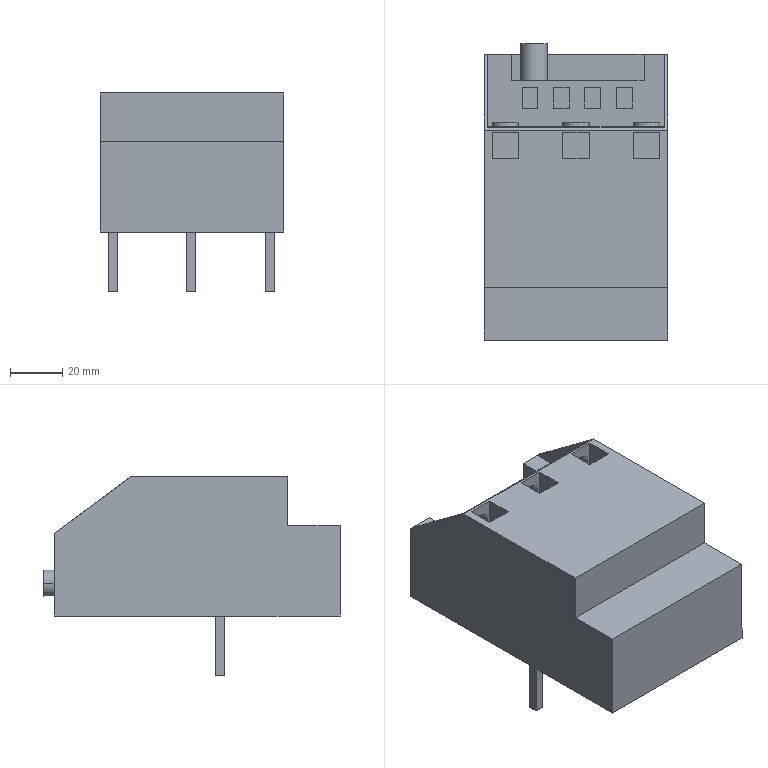Component | SolidWorks | LRD340CThermalRelaySchneider-1 | 1 solid | 124 faces | box 70 x 113 x 75.5 mm | volume 318931 mm3 | plane 93 | cylinder 31 | commonest cylinder face diameters 6 x10 10 x8 7.989 x4 7.965 x4 7.868 x4 5.967 x1
build123d program:
from build123d import *

# Parameters (mm, degrees)
BOSS_EXTRUDE1_DEPTH  = 70
SKETCH2_W            = 67.421
SKETCH2_H            = 20.48
CUT_EXTRUDE1_DEPTH   = 28
SKETCH3_R            = 4
CUT_EXTRUDE2_DEPTH   = 15
SKETCH4_R            = 5
SKETCH4_R_2          = 3.934
SKETCH4_R_3          = 3.982
SKETCH4_R_4          = 3.994
BOSS_EXTRUDE3_DEPTH  = 17
SKETCH5_W            = 10
SKETCH5_H            = 10
CUT_EXTRUDE3_DEPTH   = 15
SKETCH6_W            = 50.414
SKETCH6_H            = 31.5
CUT_EXTRUDE4_DEPTH   = 10
SKETCH7_R            = 3
CUT_EXTRUDE5_DEPTH   = 10
SKETCH9_W            = 8
SKETCH9_H            = 6
CUT_EXTRUDE6_DEPTH   = 9
SKETCH10_W           = 50.414
SKETCH10_H           = 6.044
BOSS_EXTRUDE4_DEPTH  = 10
SKETCH11_R           = 5
SKETCH11_R_2         = 3
BOSS_EXTRUDE5_DEPTH  = 14
BOSS_EXTRUDE9_DEPTH  = 14
SKETCH13_W           = 3.5
SKETCH13_H           = 3.5
BOSS_EXTRUDE10_DEPTH = 22.5


with BuildPart() as part:
    # Sketch1 → Boss-Extrude1 (new body)
    with BuildSketch(Plane.XY):
        Polygon((-34.195, 45.063), (-34.195, 10.563), (-14.195, 10.563), (-14.195, -7.937), (45.805, -7.937), (74.805, 13.563), (74.805, 45.063), align=None)
    extrude(amount=BOSS_EXTRUDE1_DEPTH)

    # Sketch2 → Cut-Extrude1 (cut)
    with BuildSketch(Plane(origin=(74.805, 0, 0), x_dir=(0, 0, -1), z_dir=(1, 0, 0))):
        with Locations((-35.046, 3.323)):
            Rectangle(SKETCH2_W, SKETCH2_H)
    extrude(amount=-CUT_EXTRUDE1_DEPTH, mode=Mode.SUBTRACT)

    # Sketch3 → Cut-Extrude2 (cut)
    with BuildSketch(Plane(origin=(46.805, 0, 0), x_dir=(0, 0, -1), z_dir=(1, 0, 0))):
        with Locations((-62, 0.06321)):
            Circle(SKETCH3_R)
        with Locations((-35, 0.06321)):
            Circle(SKETCH3_R)
        with Locations((-8, 0.06321)):
            Circle(SKETCH3_R)
    extrude(amount=-CUT_EXTRUDE2_DEPTH, mode=Mode.SUBTRACT)

    # Sketch4 → Boss-Extrude3 (add)
    # profile 1 of 3: a face of its own
    with BuildSketch(Plane(origin=(31.805, 0, 0), x_dir=(0, 0, -1), z_dir=(1, 0, 0))):
        with Locations((-62, 0.06321)):
            Circle(SKETCH4_R)
        with Locations((-62, 0.06321)):
            Circle(SKETCH4_R_2, mode=Mode.SUBTRACT)
    # profile 2 of 3: a face of its own
    with BuildSketch(Plane(origin=(31.805, 0, 0), x_dir=(0, 0, -1), z_dir=(1, 0, 0))):
        with Locations((-35, 0.06321)):
            Circle(SKETCH4_R)
        with Locations((-35, 0.06321)):
            Circle(SKETCH4_R_3, mode=Mode.SUBTRACT)
    # profile 3 of 3: a face of its own
    with BuildSketch(Plane(origin=(31.805, 0, 0), x_dir=(0, 0, -1), z_dir=(1, 0, 0))):
        with Locations((-8, 0.06321)):
            Circle(SKETCH4_R)
        with Locations((-8, 0.06321)):
            Circle(SKETCH4_R_4, mode=Mode.SUBTRACT)
    extrude(amount=BOSS_EXTRUDE3_DEPTH)

    # Sketch5 → Cut-Extrude3 (cut)
    with BuildSketch(Plane.XZ.offset(7.937)):
        with Locations((39.82, 35)):
            Rectangle(SKETCH5_W, SKETCH5_H)
        with Locations((39.82, 62)):
            Rectangle(SKETCH5_W, SKETCH5_H)
        with Locations((39.82, 8)):
            Rectangle(SKETCH5_W, SKETCH5_H)
    extrude(amount=-CUT_EXTRUDE3_DEPTH, mode=Mode.SUBTRACT)

    # Sketch6 → Cut-Extrude4 (cut)
    with BuildSketch(Plane(origin=(74.805, 0, 0), x_dir=(0, 0, -1), z_dir=(1, 0, 0))):
        with Locations((-34.279, 29.313)):
            Rectangle(SKETCH6_W, SKETCH6_H)
    extrude(amount=-CUT_EXTRUDE4_DEPTH, mode=Mode.SUBTRACT)

    # Sketch7 → Cut-Extrude5 (cut)
    with BuildSketch(Plane(origin=(64.805, 0, 0), x_dir=(0, 0, -1), z_dir=(1, 0, 0))):
        with Locations((-52.44, 18.63)):
            Circle(SKETCH7_R)
        with Locations((-40.44, 18.63)):
            Circle(SKETCH7_R)
        with Locations((-28.44, 18.63)):
            Circle(SKETCH7_R)
        with Locations((-16.44, 18.63)):
            Circle(SKETCH7_R)
    extrude(amount=-CUT_EXTRUDE5_DEPTH, mode=Mode.SUBTRACT)

    # Sketch9 → Cut-Extrude6 (cut)
    with BuildSketch(Plane.XZ.offset(-13.563)):
        with Locations((58.209, 40.574)):
            Rectangle(SKETCH9_W, SKETCH9_H)
        with Locations((58.209, 52.574)):
            Rectangle(SKETCH9_W, SKETCH9_H)
        with Locations((58.209, 28.574)):
            Rectangle(SKETCH9_W, SKETCH9_H)
        with Locations((58.209, 16.574)):
            Rectangle(SKETCH9_W, SKETCH9_H)
    extrude(amount=-CUT_EXTRUDE6_DEPTH, mode=Mode.SUBTRACT)

    # Sketch10 → Boss-Extrude4 (add)
    with BuildSketch(Plane(origin=(64.805, 0, 0), x_dir=(0, 0, -1), z_dir=(1, 0, 0))):
        with Locations((-34.279, 42.041)):
            Rectangle(SKETCH10_W, SKETCH10_H)
    extrude(amount=BOSS_EXTRUDE4_DEPTH)

    # Sketch11 → Boss-Extrude5 (add)
    with BuildSketch(Plane(origin=(64.805, 0, 0), x_dir=(0, 0, -1), z_dir=(1, 0, 0))):
        with Locations((-51.029, 32.654)):
            Circle(SKETCH11_R)
        with Locations((-51.029, 32.654)):
            Circle(SKETCH11_R_2, mode=Mode.SUBTRACT)
    extrude(amount=BOSS_EXTRUDE5_DEPTH)

    # Sketch12 → Boss-Extrude9 (add)
    with BuildSketch(Plane(origin=(64.805, 0, 0), x_dir=(0, 0, -1), z_dir=(1, 0, 0))):
        with BuildLine():
            Line((-53.837, 31.645), (-51.902, 31.645))
            Line((-51.902, 31.645), (-51.902, 29.821))
            Line((-51.902, 29.821), (-50.092, 29.821))
            Line((-50.092, 29.821), (-50.092, 31.645))
            Line((-50.092, 31.645), (-48.222, 31.645))
            Line((-48.222, 31.645), (-48.222, 33.663))
            Line((-48.222, 33.663), (-50.092, 33.663))
            Line((-50.092, 33.663), (-50.092, 35.486))
            ThreePointArc((-50.092, 35.486), (-50.124, 35.497), (-50.157, 35.507))
            Line((-50.157, 35.507), (-51.902, 35.507))
            Line((-51.902, 35.507), (-51.902, 33.663))
            Line((-51.902, 33.663), (-53.837, 33.663))
            Line((-53.837, 33.663), (-53.837, 31.645))
        make_face()
    extrude(amount=BOSS_EXTRUDE9_DEPTH)

    # Sketch13 → Boss-Extrude10 (add)
    with BuildSketch(Plane(origin=(0, 45.063, 0), x_dir=(1, 0, 0), z_dir=(0, 1, 0))):
        with Locations((11.555, -35.25)):
            Rectangle(SKETCH13_W, SKETCH13_H)
        with Locations((11.555, -65.25)):
            Rectangle(SKETCH13_W, SKETCH13_H)
        with Locations((11.555, -5.25)):
            Rectangle(SKETCH13_W, SKETCH13_H)
    extrude(amount=BOSS_EXTRUDE10_DEPTH)


solid = part.part

# Placed as in the assembly
solid = solid.moved(Location((3.893, -14.983, 1068.581), (-90, -90, 0)))